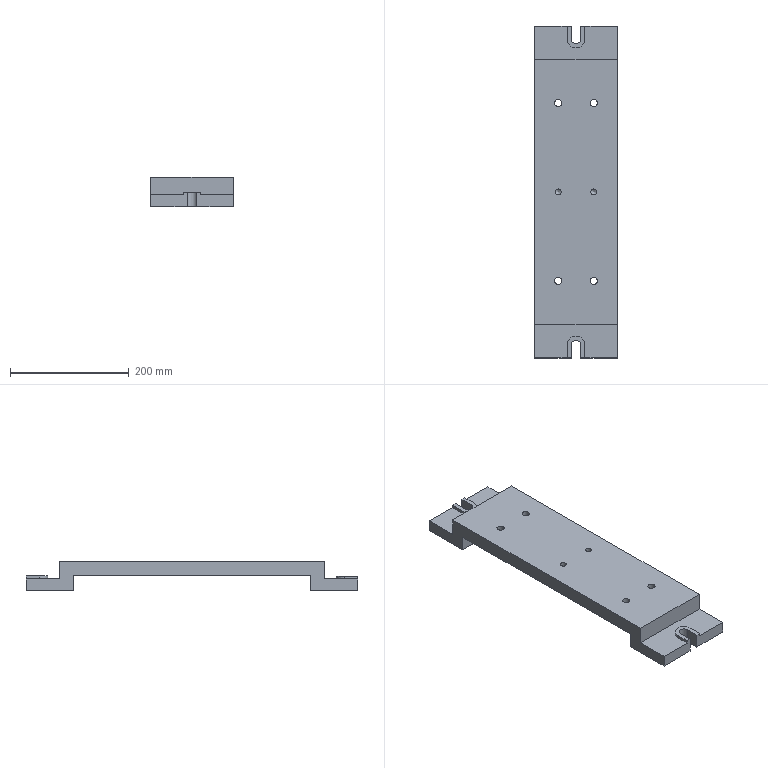Component | NX | BASE_PLATE | 1 solid | 38 faces | volume 1967737 mm3 | plane 26 | cylinder 10 | cone 2 | commonest cylinder face diameters 12 x4 10 x2 16 x2 30 x2